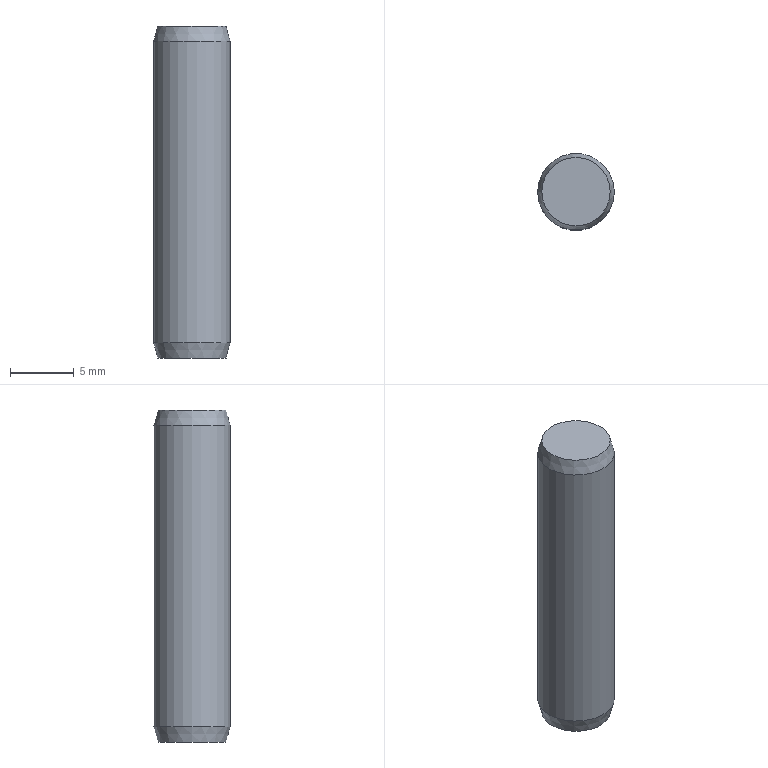Component | NX | GB-T119_1-2000_6X26_2 | 1 solid | 5 faces | box 6 x 6 x 26 mm | volume 728 mm3 | plane 2 | cone 2 | cylinder 1 | commonest cylinder face diameters 6 x1
STEP:
#1=CARTESIAN_POINT('',(0.,0.,0.));
#2=DIRECTION('',(0.,0.,1.));
#3=DIRECTION('',(1.,0.,0.));
#4=AXIS2_PLACEMENT_3D('',#1,#2,#3);
#5=CARTESIAN_POINT('',(-22.678,70.,108.5));
#6=VERTEX_POINT('',#5);
#7=CARTESIAN_POINT('',(-20.,70.,108.5));
#8=DIRECTION('',(0.,0.,-1.));
#9=DIRECTION('',(-1.,0.,0.));
#10=AXIS2_PLACEMENT_3D('',#7,#8,#9);
#11=CIRCLE('',#10,2.678);
#12=CARTESIAN_POINT('',(-20.,70.,108.5));
#13=DIRECTION('',(0.,0.,-1.));
#14=DIRECTION('',(-1.,0.,0.));
#15=AXIS2_PLACEMENT_3D('',#12,#13,#14);
#16=PLANE('',#15);
#17=CARTESIAN_POINT('',(0.,0.));
#18=DIRECTION('',(1.,0.));
#19=AXIS2_PLACEMENT_2D('',#17,#18);
#20=CIRCLE('',#19,2.678);
#21=(GEOMETRIC_REPRESENTATION_CONTEXT(2)PARAMETRIC_REPRESENTATION_CONTEXT()REPRESENTATION_CONTEXT('',''));
#22=DEFINITIONAL_REPRESENTATION('',(#20),#21);
#23=PCURVE('',#16,#22);
#24=CARTESIAN_POINT('',(-20.,70.,108.5));
#25=DIRECTION('',(0.,0.,1.));
#26=DIRECTION('',(1.,0.,0.));
#27=AXIS2_PLACEMENT_3D('',#24,#25,#26);
#28=CONICAL_SURFACE('',#27,2.678,0.2618);
#29=CARTESIAN_POINT('',(9.425,0.));
#30=DIRECTION('',(-1.,0.));
#31=VECTOR('',#30,1.);
#32=LINE('',#29,#31);
#33=(GEOMETRIC_REPRESENTATION_CONTEXT(2)PARAMETRIC_REPRESENTATION_CONTEXT()REPRESENTATION_CONTEXT('',''));
#34=DEFINITIONAL_REPRESENTATION('',(#32),#33);
#35=PCURVE('',#28,#34);
#36=SURFACE_CURVE('',#11,(#23,#35),.PCURVE_S1.);
#37=EDGE_CURVE('',#6,#6,#36,.T.);
#38=ORIENTED_EDGE('',*,*,#37,.T.);
#39=EDGE_LOOP('',(#38));
#40=FACE_BOUND('',#39,.T.);
#41=ADVANCED_FACE('',(#40),#16,.T.);
#42=CARTESIAN_POINT('',(-23.,70.,109.7));
#43=VERTEX_POINT('',#42);
#44=CARTESIAN_POINT('',(-20.,70.,109.7));
#45=DIRECTION('',(0.,0.,-1.));
#46=DIRECTION('',(-1.,0.,0.));
#47=AXIS2_PLACEMENT_3D('',#44,#45,#46);
#48=CIRCLE('',#47,3.);
#49=CARTESIAN_POINT('',(9.425,1.2));
#50=DIRECTION('',(-1.,0.));
#51=VECTOR('',#50,1.);
#52=LINE('',#49,#51);
#53=(GEOMETRIC_REPRESENTATION_CONTEXT(2)PARAMETRIC_REPRESENTATION_CONTEXT()REPRESENTATION_CONTEXT('',''));
#54=DEFINITIONAL_REPRESENTATION('',(#52),#53);
#55=PCURVE('',#28,#54);
#56=CARTESIAN_POINT('',(-20.,70.,134.5));
#57=DIRECTION('',(0.,0.,-1.));
#58=DIRECTION('',(-1.,0.,0.));
#59=AXIS2_PLACEMENT_3D('',#56,#57,#58);
#60=CYLINDRICAL_SURFACE('',#59,3.);
#61=CARTESIAN_POINT('',(0.,24.8));
#62=DIRECTION('',(1.,0.));
#63=VECTOR('',#62,1.);
#64=LINE('',#61,#63);
#65=(GEOMETRIC_REPRESENTATION_CONTEXT(2)PARAMETRIC_REPRESENTATION_CONTEXT()REPRESENTATION_CONTEXT('',''));
#66=DEFINITIONAL_REPRESENTATION('',(#64),#65);
#67=PCURVE('',#60,#66);
#68=SURFACE_CURVE('',#48,(#55,#67),.PCURVE_S1.);
#69=EDGE_CURVE('',#43,#43,#68,.T.);
#70=ORIENTED_EDGE('',*,*,#69,.T.);
#71=CARTESIAN_POINT('',(-22.678,70.,108.5));
#72=CARTESIAN_POINT('',(-23.,70.,109.7));
#73=B_SPLINE_CURVE_WITH_KNOTS('',1,(#71,#72),.UNSPECIFIED.,.F.,.F.,(2,2),(0.,1.242),.PIECEWISE_BEZIER_KNOTS.);
#74=CARTESIAN_POINT('',(3.142,0.));
#75=DIRECTION('',(0.,1.));
#76=VECTOR('',#75,1.);
#77=LINE('',#74,#76);
#78=(GEOMETRIC_REPRESENTATION_CONTEXT(2)PARAMETRIC_REPRESENTATION_CONTEXT()REPRESENTATION_CONTEXT('',''));
#79=DEFINITIONAL_REPRESENTATION('',(#77),#78);
#80=PCURVE('',#28,#79);
#81=CARTESIAN_POINT('',(9.425,0.));
#82=DIRECTION('',(0.,1.));
#83=VECTOR('',#82,1.);
#84=LINE('',#81,#83);
#85=(GEOMETRIC_REPRESENTATION_CONTEXT(2)PARAMETRIC_REPRESENTATION_CONTEXT()REPRESENTATION_CONTEXT('',''));
#86=DEFINITIONAL_REPRESENTATION('',(#84),#85);
#87=PCURVE('',#28,#86);
#88=SEAM_CURVE('',#73,(#80,#87),.PCURVE_S1.);
#89=EDGE_CURVE('',#6,#43,#88,.T.);
#90=ORIENTED_EDGE('',*,*,#89,.F.);
#91=ORIENTED_EDGE('',*,*,#37,.F.);
#92=ORIENTED_EDGE('',*,*,#89,.T.);
#93=EDGE_LOOP('',(#70,#90,#91,#92));
#94=FACE_BOUND('',#93,.T.);
#95=ADVANCED_FACE('',(#94),#28,.T.);
#96=CARTESIAN_POINT('',(-23.,70.,133.3));
#97=VERTEX_POINT('',#96);
#98=CARTESIAN_POINT('',(-20.,70.,133.3));
#99=DIRECTION('',(0.,0.,-1.));
#100=DIRECTION('',(-1.,0.,0.));
#101=AXIS2_PLACEMENT_3D('',#98,#99,#100);
#102=CIRCLE('',#101,3.);
#103=CARTESIAN_POINT('',(0.,1.2));
#104=DIRECTION('',(1.,0.));
#105=VECTOR('',#104,1.);
#106=LINE('',#103,#105);
#107=(GEOMETRIC_REPRESENTATION_CONTEXT(2)PARAMETRIC_REPRESENTATION_CONTEXT()REPRESENTATION_CONTEXT('',''));
#108=DEFINITIONAL_REPRESENTATION('',(#106),#107);
#109=PCURVE('',#60,#108);
#110=CARTESIAN_POINT('',(-20.,70.,133.3));
#111=DIRECTION('',(0.,0.,-1.));
#112=DIRECTION('',(-1.,0.,0.));
#113=AXIS2_PLACEMENT_3D('',#110,#111,#112);
#114=CONICAL_SURFACE('',#113,3.,0.2618);
#115=CARTESIAN_POINT('',(0.,0.));
#116=DIRECTION('',(1.,0.));
#117=VECTOR('',#116,1.);
#118=LINE('',#115,#117);
#119=(GEOMETRIC_REPRESENTATION_CONTEXT(2)PARAMETRIC_REPRESENTATION_CONTEXT()REPRESENTATION_CONTEXT('',''));
#120=DEFINITIONAL_REPRESENTATION('',(#118),#119);
#121=PCURVE('',#114,#120);
#122=SURFACE_CURVE('',#102,(#109,#121),.PCURVE_S1.);
#123=EDGE_CURVE('',#97,#97,#122,.T.);
#124=ORIENTED_EDGE('',*,*,#123,.T.);
#125=CARTESIAN_POINT('',(-23.,70.,133.3));
#126=CARTESIAN_POINT('',(-23.,70.,109.7));
#127=B_SPLINE_CURVE_WITH_KNOTS('',1,(#125,#126),.UNSPECIFIED.,.F.,.F.,(2,2),(1.2,24.8),.PIECEWISE_BEZIER_KNOTS.);
#128=CARTESIAN_POINT('',(6.283,0.));
#129=DIRECTION('',(0.,1.));
#130=VECTOR('',#129,1.);
#131=LINE('',#128,#130);
#132=(GEOMETRIC_REPRESENTATION_CONTEXT(2)PARAMETRIC_REPRESENTATION_CONTEXT()REPRESENTATION_CONTEXT('',''));
#133=DEFINITIONAL_REPRESENTATION('',(#131),#132);
#134=PCURVE('',#60,#133);
#135=CARTESIAN_POINT('',(0.,0.));
#136=DIRECTION('',(0.,1.));
#137=VECTOR('',#136,1.);
#138=LINE('',#135,#137);
#139=(GEOMETRIC_REPRESENTATION_CONTEXT(2)PARAMETRIC_REPRESENTATION_CONTEXT()REPRESENTATION_CONTEXT('',''));
#140=DEFINITIONAL_REPRESENTATION('',(#138),#139);
#141=PCURVE('',#60,#140);
#142=SEAM_CURVE('',#127,(#134,#141),.PCURVE_S1.);
#143=EDGE_CURVE('',#97,#43,#142,.T.);
#144=ORIENTED_EDGE('',*,*,#143,.T.);
#145=ORIENTED_EDGE('',*,*,#69,.F.);
#146=ORIENTED_EDGE('',*,*,#143,.F.);
#147=EDGE_LOOP('',(#124,#144,#145,#146));
#148=FACE_BOUND('',#147,.T.);
#149=ADVANCED_FACE('',(#148),#60,.T.);
#150=CARTESIAN_POINT('',(-22.678,70.,134.5));
#151=VERTEX_POINT('',#150);
#152=CARTESIAN_POINT('',(-20.,70.,134.5));
#153=DIRECTION('',(0.,0.,-1.));
#154=DIRECTION('',(-1.,0.,0.));
#155=AXIS2_PLACEMENT_3D('',#152,#153,#154);
#156=CIRCLE('',#155,2.678);
#157=CARTESIAN_POINT('',(0.,-1.2));
#158=DIRECTION('',(1.,0.));
#159=VECTOR('',#158,1.);
#160=LINE('',#157,#159);
#161=(GEOMETRIC_REPRESENTATION_CONTEXT(2)PARAMETRIC_REPRESENTATION_CONTEXT()REPRESENTATION_CONTEXT('',''));
#162=DEFINITIONAL_REPRESENTATION('',(#160),#161);
#163=PCURVE('',#114,#162);
#164=CARTESIAN_POINT('',(-17.322,70.,134.5));
#165=DIRECTION('',(0.,0.,1.));
#166=DIRECTION('',(1.,0.,0.));
#167=AXIS2_PLACEMENT_3D('',#164,#165,#166);
#168=PLANE('',#167);
#169=CARTESIAN_POINT('',(-5.357,0.));
#170=CARTESIAN_POINT('',(-5.357,4.639));
#171=CARTESIAN_POINT('',(-1.339,2.32));
#172=CARTESIAN_POINT('',(2.678,0.));
#173=CARTESIAN_POINT('',(-1.339,-2.32));
#174=CARTESIAN_POINT('',(-5.357,-4.639));
#175=CARTESIAN_POINT('',(-5.357,0.));
#176=(BOUNDED_CURVE()B_SPLINE_CURVE(2,(#169,#170,#171,#172,#173,#174,#175),.UNSPECIFIED.,.T.,.F.)B_SPLINE_CURVE_WITH_KNOTS((1,2,2,2,2,1),(-2.094,0.,2.094,4.189,6.283,8.378),.UNSPECIFIED.)CURVE()GEOMETRIC_REPRESENTATION_ITEM()RATIONAL_B_SPLINE_CURVE((1.,0.5,1.,0.5,1.,0.5,1.))REPRESENTATION_ITEM(''));
#177=(GEOMETRIC_REPRESENTATION_CONTEXT(2)PARAMETRIC_REPRESENTATION_CONTEXT()REPRESENTATION_CONTEXT('',''));
#178=DEFINITIONAL_REPRESENTATION('',(#176),#177);
#179=PCURVE('',#168,#178);
#180=SURFACE_CURVE('',#156,(#163,#179),.PCURVE_S1.);
#181=EDGE_CURVE('',#151,#151,#180,.T.);
#182=ORIENTED_EDGE('',*,*,#181,.T.);
#183=CARTESIAN_POINT('',(-22.678,70.,134.5));
#184=CARTESIAN_POINT('',(-23.,70.,133.3));
#185=B_SPLINE_CURVE_WITH_KNOTS('',1,(#183,#184),.UNSPECIFIED.,.F.,.F.,(2,2),(-1.242,0.),.PIECEWISE_BEZIER_KNOTS.);
#186=CARTESIAN_POINT('',(6.283,0.));
#187=DIRECTION('',(0.,1.));
#188=VECTOR('',#187,1.);
#189=LINE('',#186,#188);
#190=(GEOMETRIC_REPRESENTATION_CONTEXT(2)PARAMETRIC_REPRESENTATION_CONTEXT()REPRESENTATION_CONTEXT('',''));
#191=DEFINITIONAL_REPRESENTATION('',(#189),#190);
#192=PCURVE('',#114,#191);
#193=CARTESIAN_POINT('',(0.,0.));
#194=DIRECTION('',(0.,1.));
#195=VECTOR('',#194,1.);
#196=LINE('',#193,#195);
#197=(GEOMETRIC_REPRESENTATION_CONTEXT(2)PARAMETRIC_REPRESENTATION_CONTEXT()REPRESENTATION_CONTEXT('',''));
#198=DEFINITIONAL_REPRESENTATION('',(#196),#197);
#199=PCURVE('',#114,#198);
#200=SEAM_CURVE('',#185,(#192,#199),.PCURVE_S1.);
#201=EDGE_CURVE('',#151,#97,#200,.T.);
#202=ORIENTED_EDGE('',*,*,#201,.T.);
#203=ORIENTED_EDGE('',*,*,#123,.F.);
#204=ORIENTED_EDGE('',*,*,#201,.F.);
#205=EDGE_LOOP('',(#182,#202,#203,#204));
#206=FACE_BOUND('',#205,.T.);
#207=ADVANCED_FACE('',(#206),#114,.T.);
#208=ORIENTED_EDGE('',*,*,#181,.F.);
#209=EDGE_LOOP('',(#208));
#210=FACE_BOUND('',#209,.T.);
#211=ADVANCED_FACE('',(#210),#168,.T.);
#212=CLOSED_SHELL('',(#41,#95,#149,#207,#211));
#213=MANIFOLD_SOLID_BREP('',#212);
#214=(LENGTH_UNIT()NAMED_UNIT(*)SI_UNIT(.MILLI.,.METRE.));
#215=UNCERTAINTY_MEASURE_WITH_UNIT(LENGTH_MEASURE(0.00001),#214,'','');
#216=(NAMED_UNIT(*)PLANE_ANGLE_UNIT()SI_UNIT($,.RADIAN.));
#217=(NAMED_UNIT(*)SI_UNIT($,.STERADIAN.)SOLID_ANGLE_UNIT());
#218=(GEOMETRIC_REPRESENTATION_CONTEXT(3)GLOBAL_UNCERTAINTY_ASSIGNED_CONTEXT((#215))GLOBAL_UNIT_ASSIGNED_CONTEXT((#214,#216,#217))REPRESENTATION_CONTEXT('',''));
#219=ADVANCED_BREP_SHAPE_REPRESENTATION('',(#4,#213),#218);